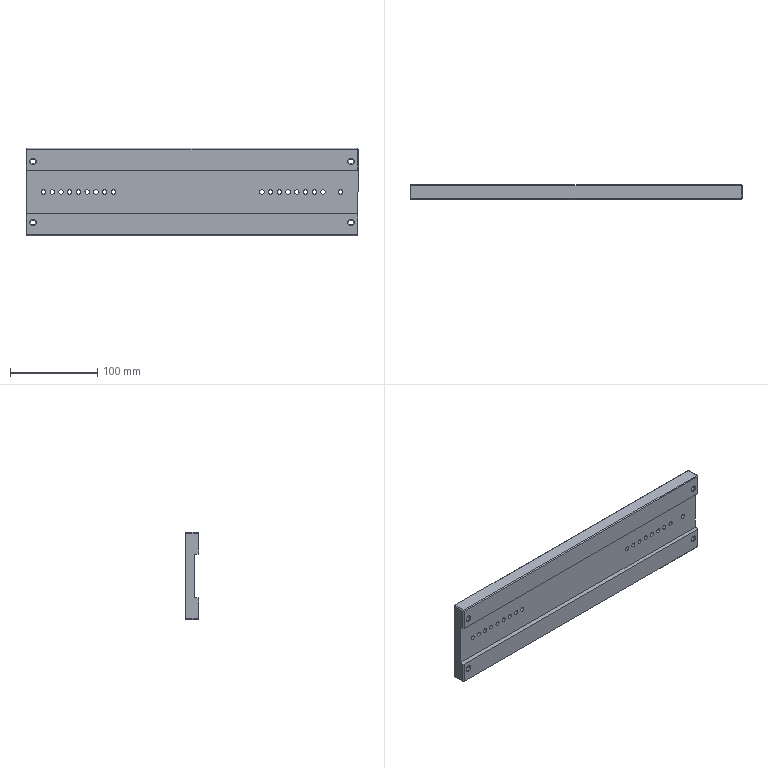Component | SolidWorks | GuidePlate-1 | 1 solid | 84 faces | box 380 x 16 x 100 mm | volume 506578 mm3 | cylinder 44 | plane 24 | cone 16 | commonest cylinder face diameters 5 x36 5.5 x8
build123d program:
from build123d import *

# Parameters (mm, degrees)
SKETCH1_W           = 380
SKETCH1_H           = 100
SKETCH1_R           = 2.75
BOSS_EXTRUDE1_DEPTH = 16
CHAMFER1_SIZE       = 1
CHAMFER2_SIZE       = 1
CHAMFER3_SIZE       = 1
M6_TAPPED_HOLE1_D   = 5
SKETCH4_W           = 6.757
SKETCH4_H           = 50
CUT_EXTRUDE1_DEPTH  = 394.263


with BuildPart() as part:
    # Sketch1 → Boss-Extrude1 (new body)
    with BuildSketch(Plane.XY):
        with Locations((190, -50)):
            Rectangle(SKETCH1_W, SKETCH1_H)
        with Locations((8, -15)):
            Circle(SKETCH1_R, mode=Mode.SUBTRACT)
        with Locations((8, -85)):
            Circle(SKETCH1_R, mode=Mode.SUBTRACT)
        with Locations((372, -15)):
            Circle(SKETCH1_R, mode=Mode.SUBTRACT)
        with Locations((372, -85)):
            Circle(SKETCH1_R, mode=Mode.SUBTRACT)
    extrude(amount=BOSS_EXTRUDE1_DEPTH)

    # Chamfer1
    chamfer1_edges = [part.edges().sort_by_distance(p)[0] for p in [
        (5.25, -15, 0),
        (5.25, -85, 0),
        (369.25, -15, 0),
        (369.25, -85, 0),
        (190, 0, 0),
        (380, -50, 0),
        (190, -100, 0),
        (0, -50, 0),
    ]]
    chamfer(chamfer1_edges, length=CHAMFER1_SIZE)

    # Chamfer2
    chamfer2_edges = [part.edges().sort_by_distance(p)[0] for p in [
        (380, -50, 16),
        (5.25, -15, 16),
        (190, 0, 16),
        (5.25, -85, 16),
        (369.25, -15, 16),
        (369.25, -85, 16),
        (0, -50, 16),
        (190, -100, 16),
    ]]
    chamfer(chamfer2_edges, length=CHAMFER2_SIZE)

    # Chamfer3
    chamfer3_edges = [part.edges().sort_by_distance(p)[0] for p in [
        (380, 0, 8),
        (0, 0, 8),
        (380, -100, 8),
        (0, -100, 8),
    ]]
    chamfer(chamfer3_edges, length=CHAMFER3_SIZE)

    # M6 Tapped Hole1 (through all)
    with Locations(Plane(origin=(0, 0, 0), x_dir=(-1, 0, 0), z_dir=(0, 0, -1))):
        with Locations((-360, -50), (-340, -50), (-320, -50), (-300, -50), (-280, -50), (-20, -50), (-40, -50), (-60, -50), (-80, -50), (-100, -50), (-330, -50), (-310, -50), (-290, -50), (-270, -50), (-90, -50), (-70, -50), (-50, -50), (-30, -50)):
            Hole(M6_TAPPED_HOLE1_D / 2)

    # Sketch4 → Cut-Extrude1 (cut, through all)
    with BuildSketch(Plane(origin=(380, 0, 0), x_dir=(0, 0, -1), z_dir=(1, 0, 0))):
        with Locations((-1.621, -50)):
            Rectangle(SKETCH4_W, SKETCH4_H)
    extrude(amount=-CUT_EXTRUDE1_DEPTH, mode=Mode.SUBTRACT)


solid = part.part

# Placed as in the assembly
solid = solid.moved(Location((-367.951, 421.323, -325), (-90, 0, 0)))